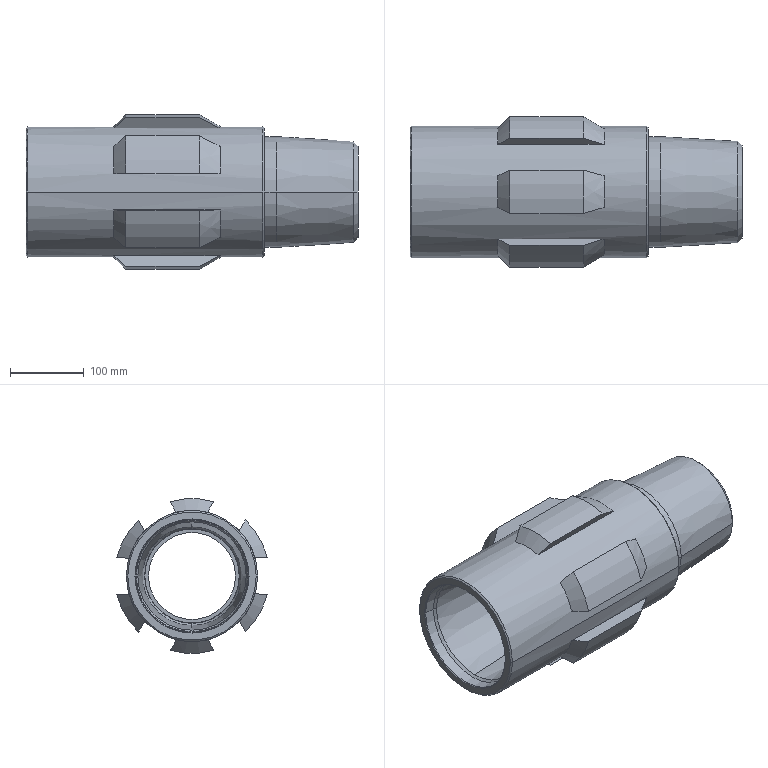Component | SolidWorks | 216OuterTube-1_LowerCentralizer-1 | 1 solid | 64 faces | volume 5067345 mm3 | cone 34 | plane 16 | cylinder 14 | commonest cylinder face diameters 210 x6 178 x2 150 x2 118 x2 128 x2 | material Alloy Steel